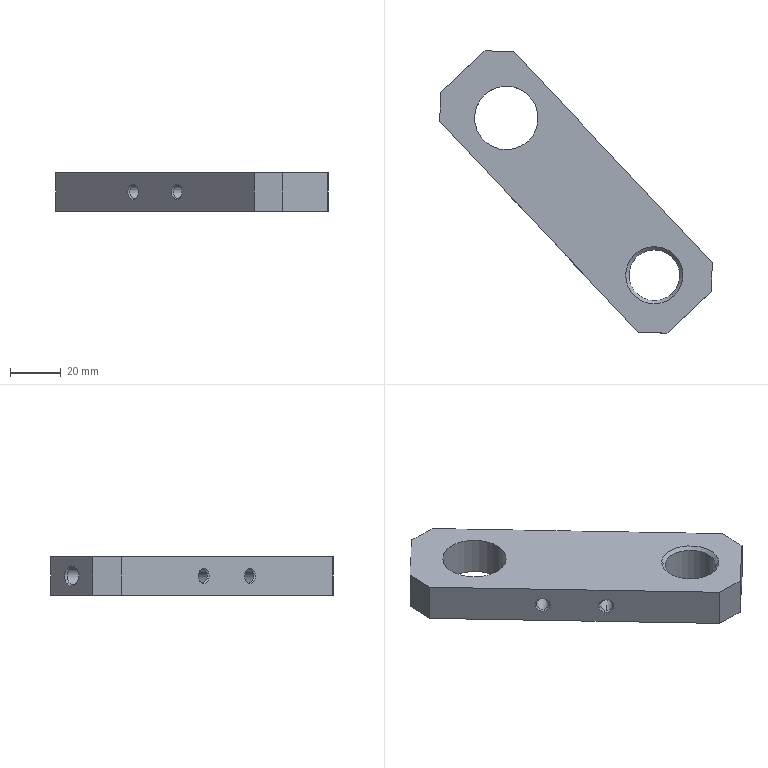Component | SolidWorks | LeftSupportBlock-1 | 1 solid | 32 faces | box 107.26 x 111.11 x 15 mm | volume 62679 mm3 | cone 12 | cylinder 10 | plane 10 | commonest cylinder face diameters 5 x4 6.8 x2 25 x2 20 x2
STEP:
#1=COLOUR_RGB('',0.7922,0.8196,0.9333);
#2=FILL_AREA_STYLE_COLOUR('',#1);
#3=FILL_AREA_STYLE('',(#2));
#4=SURFACE_STYLE_FILL_AREA(#3);
#5=SURFACE_SIDE_STYLE('',(#4));
#6=SURFACE_STYLE_USAGE(.BOTH.,#5);
#7=PRESENTATION_STYLE_ASSIGNMENT((#6));
#8=CARTESIAN_POINT('',(12.703,20.379,9.657));
#9=VERTEX_POINT('',#8);
#10=CARTESIAN_POINT('',(12.703,20.379,9.461));
#11=VERTEX_POINT('',#10);
#12=CARTESIAN_POINT('',(12.703,20.379,9.559));
#13=DIRECTION('',(-0.7282,-0.6854,-0.));
#14=DIRECTION('',(0.,0.,-1.));
#15=AXIS2_PLACEMENT_3D('',#12,#13,#14);
#16=CIRCLE('',#15,0.09843);
#17=EDGE_CURVE('',#9,#11,#16,.T.);
#18=ORIENTED_EDGE('',*,*,#17,.F.);
#19=CARTESIAN_POINT('',(12.688,20.365,9.678));
#20=VERTEX_POINT('',#19);
#21=CARTESIAN_POINT('',(12.688,20.365,9.678));
#22=DIRECTION('',(-0.5149,-0.4846,0.7071));
#23=VECTOR('',#22,39.37);
#24=LINE('',#21,#23);
#25=EDGE_CURVE('',#9,#20,#24,.T.);
#26=ORIENTED_EDGE('',*,*,#25,.T.);
#27=CARTESIAN_POINT('',(12.688,20.365,9.44));
#28=VERTEX_POINT('',#27);
#29=CARTESIAN_POINT('',(12.688,20.365,9.559));
#30=DIRECTION('',(-0.7282,-0.6854,-0.));
#31=DIRECTION('',(0.,0.,-1.));
#32=AXIS2_PLACEMENT_3D('',#29,#30,#31);
#33=CIRCLE('',#32,0.1191);
#34=EDGE_CURVE('',#20,#28,#33,.T.);
#35=ORIENTED_EDGE('',*,*,#34,.T.);
#36=CARTESIAN_POINT('',(12.688,20.365,9.44));
#37=DIRECTION('',(-0.5149,-0.4846,-0.7071));
#38=VECTOR('',#37,39.37);
#39=LINE('',#36,#38);
#40=EDGE_CURVE('',#11,#28,#39,.T.);
#41=ORIENTED_EDGE('',*,*,#40,.F.);
#42=EDGE_LOOP('',(#18,#26,#35,#41));
#43=FACE_OUTER_BOUND('',#42,.T.);
#44=CARTESIAN_POINT('',(12.688,20.365,9.559));
#45=DIRECTION('',(-0.7282,-0.6854,-0.));
#46=DIRECTION('',(0.,0.,-1.));
#47=AXIS2_PLACEMENT_3D('',#44,#45,#46);
#48=CONICAL_SURFACE('',#47,0.1191,0.7854);
#49=ADVANCED_FACE('',(#43),#48,.F.);
#50=CARTESIAN_POINT('',(13.262,20.905,9.657));
#51=VERTEX_POINT('',#50);
#52=CARTESIAN_POINT('',(13.262,20.905,9.461));
#53=VERTEX_POINT('',#52);
#54=CARTESIAN_POINT('',(13.262,20.905,9.559));
#55=DIRECTION('',(-0.7282,-0.6854,-0.));
#56=DIRECTION('',(0.,0.,-1.));
#57=AXIS2_PLACEMENT_3D('',#54,#55,#56);
#58=CIRCLE('',#57,0.09843);
#59=EDGE_CURVE('',#51,#53,#58,.T.);
#60=ORIENTED_EDGE('',*,*,#59,.F.);
#61=CARTESIAN_POINT('',(12.688,20.365,9.657));
#62=DIRECTION('',(-0.7282,-0.6854,-0.));
#63=VECTOR('',#62,39.37);
#64=LINE('',#61,#63);
#65=EDGE_CURVE('',#51,#9,#64,.T.);
#66=ORIENTED_EDGE('',*,*,#65,.T.);
#67=ORIENTED_EDGE('',*,*,#17,.T.);
#68=CARTESIAN_POINT('',(12.688,20.365,9.461));
#69=DIRECTION('',(-0.7282,-0.6854,-0.));
#70=VECTOR('',#69,39.37);
#71=LINE('',#68,#70);
#72=EDGE_CURVE('',#53,#11,#71,.T.);
#73=ORIENTED_EDGE('',*,*,#72,.F.);
#74=EDGE_LOOP('',(#60,#66,#67,#73));
#75=FACE_OUTER_BOUND('',#74,.T.);
#76=CARTESIAN_POINT('',(12.688,20.365,9.559));
#77=DIRECTION('',(-0.7282,-0.6854,-0.));
#78=DIRECTION('',(0.,0.,-1.));
#79=AXIS2_PLACEMENT_3D('',#76,#77,#78);
#80=CYLINDRICAL_SURFACE('',#79,0.09843);
#81=ADVANCED_FACE('',(#75),#80,.F.);
#82=CARTESIAN_POINT('',(13.305,20.945,9.559));
#83=VERTEX_POINT('',#82);
#84=CARTESIAN_POINT('',(13.262,20.905,9.461));
#85=DIRECTION('',(-0.375,-0.353,-0.8572));
#86=VECTOR('',#85,39.37);
#87=LINE('',#84,#86);
#88=EDGE_CURVE('',#83,#53,#87,.T.);
#89=ORIENTED_EDGE('',*,*,#88,.F.);
#90=CARTESIAN_POINT('',(13.262,20.905,9.657));
#91=DIRECTION('',(-0.375,-0.353,0.8572));
#92=VECTOR('',#91,39.37);
#93=LINE('',#90,#92);
#94=EDGE_CURVE('',#83,#51,#93,.T.);
#95=ORIENTED_EDGE('',*,*,#94,.T.);
#96=ORIENTED_EDGE('',*,*,#59,.T.);
#97=EDGE_LOOP('',(#89,#95,#96));
#98=FACE_OUTER_BOUND('',#97,.T.);
#99=CARTESIAN_POINT('',(13.262,20.905,9.559));
#100=DIRECTION('',(-0.7282,-0.6854,-0.));
#101=DIRECTION('',(0.,0.,-1.));
#102=AXIS2_PLACEMENT_3D('',#99,#100,#101);
#103=CONICAL_SURFACE('',#102,0.09843,1.03);
#104=ADVANCED_FACE('',(#98),#103,.F.);
#105=CARTESIAN_POINT('',(13.378,19.662,9.657));
#106=VERTEX_POINT('',#105);
#107=CARTESIAN_POINT('',(13.378,19.662,9.461));
#108=VERTEX_POINT('',#107);
#109=CARTESIAN_POINT('',(13.378,19.662,9.559));
#110=DIRECTION('',(-0.7282,-0.6854,-0.));
#111=DIRECTION('',(0.,0.,-1.));
#112=AXIS2_PLACEMENT_3D('',#109,#110,#111);
#113=CIRCLE('',#112,0.09843);
#114=EDGE_CURVE('',#106,#108,#113,.T.);
#115=ORIENTED_EDGE('',*,*,#114,.F.);
#116=CARTESIAN_POINT('',(13.363,19.648,9.678));
#117=VERTEX_POINT('',#116);
#118=CARTESIAN_POINT('',(13.363,19.648,9.678));
#119=DIRECTION('',(-0.5149,-0.4846,0.7071));
#120=VECTOR('',#119,39.37);
#121=LINE('',#118,#120);
#122=EDGE_CURVE('',#106,#117,#121,.T.);
#123=ORIENTED_EDGE('',*,*,#122,.T.);
#124=CARTESIAN_POINT('',(13.363,19.648,9.44));
#125=VERTEX_POINT('',#124);
#126=CARTESIAN_POINT('',(13.363,19.648,9.559));
#127=DIRECTION('',(-0.7282,-0.6854,-0.));
#128=DIRECTION('',(0.,0.,-1.));
#129=AXIS2_PLACEMENT_3D('',#126,#127,#128);
#130=CIRCLE('',#129,0.1191);
#131=EDGE_CURVE('',#117,#125,#130,.T.);
#132=ORIENTED_EDGE('',*,*,#131,.T.);
#133=CARTESIAN_POINT('',(13.363,19.648,9.44));
#134=DIRECTION('',(-0.5149,-0.4846,-0.7071));
#135=VECTOR('',#134,39.37);
#136=LINE('',#133,#135);
#137=EDGE_CURVE('',#108,#125,#136,.T.);
#138=ORIENTED_EDGE('',*,*,#137,.F.);
#139=EDGE_LOOP('',(#115,#123,#132,#138));
#140=FACE_OUTER_BOUND('',#139,.T.);
#141=CARTESIAN_POINT('',(13.363,19.648,9.559));
#142=DIRECTION('',(-0.7282,-0.6854,-0.));
#143=DIRECTION('',(0.,0.,-1.));
#144=AXIS2_PLACEMENT_3D('',#141,#142,#143);
#145=CONICAL_SURFACE('',#144,0.1191,0.7854);
#146=ADVANCED_FACE('',(#140),#145,.F.);
#147=CARTESIAN_POINT('',(13.936,20.188,9.657));
#148=VERTEX_POINT('',#147);
#149=CARTESIAN_POINT('',(13.936,20.188,9.461));
#150=VERTEX_POINT('',#149);
#151=CARTESIAN_POINT('',(13.936,20.188,9.559));
#152=DIRECTION('',(-0.7282,-0.6854,-0.));
#153=DIRECTION('',(0.,0.,-1.));
#154=AXIS2_PLACEMENT_3D('',#151,#152,#153);
#155=CIRCLE('',#154,0.09843);
#156=EDGE_CURVE('',#148,#150,#155,.T.);
#157=ORIENTED_EDGE('',*,*,#156,.F.);
#158=CARTESIAN_POINT('',(13.363,19.648,9.657));
#159=DIRECTION('',(-0.7282,-0.6854,-0.));
#160=VECTOR('',#159,39.37);
#161=LINE('',#158,#160);
#162=EDGE_CURVE('',#148,#106,#161,.T.);
#163=ORIENTED_EDGE('',*,*,#162,.T.);
#164=ORIENTED_EDGE('',*,*,#114,.T.);
#165=CARTESIAN_POINT('',(13.363,19.648,9.461));
#166=DIRECTION('',(-0.7282,-0.6854,-0.));
#167=VECTOR('',#166,39.37);
#168=LINE('',#165,#167);
#169=EDGE_CURVE('',#150,#108,#168,.T.);
#170=ORIENTED_EDGE('',*,*,#169,.F.);
#171=EDGE_LOOP('',(#157,#163,#164,#170));
#172=FACE_OUTER_BOUND('',#171,.T.);
#173=CARTESIAN_POINT('',(13.363,19.648,9.559));
#174=DIRECTION('',(-0.7282,-0.6854,-0.));
#175=DIRECTION('',(0.,0.,-1.));
#176=AXIS2_PLACEMENT_3D('',#173,#174,#175);
#177=CYLINDRICAL_SURFACE('',#176,0.09843);
#178=ADVANCED_FACE('',(#172),#177,.F.);
#179=CARTESIAN_POINT('',(13.979,20.228,9.559));
#180=VERTEX_POINT('',#179);
#181=CARTESIAN_POINT('',(13.936,20.188,9.461));
#182=DIRECTION('',(-0.375,-0.353,-0.8572));
#183=VECTOR('',#182,39.37);
#184=LINE('',#181,#183);
#185=EDGE_CURVE('',#180,#150,#184,.T.);
#186=ORIENTED_EDGE('',*,*,#185,.F.);
#187=CARTESIAN_POINT('',(13.936,20.188,9.657));
#188=DIRECTION('',(-0.375,-0.353,0.8572));
#189=VECTOR('',#188,39.37);
#190=LINE('',#187,#189);
#191=EDGE_CURVE('',#180,#148,#190,.T.);
#192=ORIENTED_EDGE('',*,*,#191,.T.);
#193=ORIENTED_EDGE('',*,*,#156,.T.);
#194=EDGE_LOOP('',(#186,#192,#193));
#195=FACE_OUTER_BOUND('',#194,.T.);
#196=CARTESIAN_POINT('',(13.936,20.188,9.559));
#197=DIRECTION('',(-0.7282,-0.6854,-0.));
#198=DIRECTION('',(0.,0.,-1.));
#199=AXIS2_PLACEMENT_3D('',#196,#197,#198);
#200=CONICAL_SURFACE('',#199,0.09843,1.03);
#201=ADVANCED_FACE('',(#195),#200,.F.);
#202=CARTESIAN_POINT('',(11.862,22.392,9.425));
#203=VERTEX_POINT('',#202);
#204=CARTESIAN_POINT('',(11.862,22.392,9.693));
#205=VERTEX_POINT('',#204);
#206=CARTESIAN_POINT('',(11.862,22.392,9.559));
#207=DIRECTION('',(-0.6854,0.7282,-0.));
#208=DIRECTION('',(0.,0.,1.));
#209=AXIS2_PLACEMENT_3D('',#206,#207,#208);
#210=CIRCLE('',#209,0.1339);
#211=EDGE_CURVE('',#203,#205,#210,.T.);
#212=ORIENTED_EDGE('',*,*,#211,.F.);
#213=CARTESIAN_POINT('',(11.845,22.41,9.401));
#214=VERTEX_POINT('',#213);
#215=CARTESIAN_POINT('',(11.845,22.41,9.401));
#216=DIRECTION('',(-0.4846,0.5149,-0.7071));
#217=VECTOR('',#216,39.37);
#218=LINE('',#215,#217);
#219=EDGE_CURVE('',#203,#214,#218,.T.);
#220=ORIENTED_EDGE('',*,*,#219,.T.);
#221=CARTESIAN_POINT('',(11.845,22.41,9.718));
#222=VERTEX_POINT('',#221);
#223=CARTESIAN_POINT('',(11.845,22.41,9.559));
#224=DIRECTION('',(-0.6854,0.7282,-0.));
#225=DIRECTION('',(0.,0.,1.));
#226=AXIS2_PLACEMENT_3D('',#223,#224,#225);
#227=CIRCLE('',#226,0.1585);
#228=EDGE_CURVE('',#214,#222,#227,.T.);
#229=ORIENTED_EDGE('',*,*,#228,.T.);
#230=CARTESIAN_POINT('',(11.845,22.41,9.718));
#231=DIRECTION('',(-0.4846,0.5149,0.7071));
#232=VECTOR('',#231,39.37);
#233=LINE('',#230,#232);
#234=EDGE_CURVE('',#205,#222,#233,.T.);
#235=ORIENTED_EDGE('',*,*,#234,.F.);
#236=EDGE_LOOP('',(#212,#220,#229,#235));
#237=FACE_OUTER_BOUND('',#236,.T.);
#238=CARTESIAN_POINT('',(11.845,22.41,9.559));
#239=DIRECTION('',(-0.6854,0.7282,-0.));
#240=DIRECTION('',(0.,0.,1.));
#241=AXIS2_PLACEMENT_3D('',#238,#239,#240);
#242=CONICAL_SURFACE('',#241,0.1585,0.7854);
#243=ADVANCED_FACE('',(#237),#242,.F.);
#244=CARTESIAN_POINT('',(12.182,22.051,9.425));
#245=VERTEX_POINT('',#244);
#246=CARTESIAN_POINT('',(12.182,22.051,9.693));
#247=VERTEX_POINT('',#246);
#248=CARTESIAN_POINT('',(12.182,22.051,9.425));
#249=CARTESIAN_POINT('',(12.176,22.045,9.425));
#250=CARTESIAN_POINT('',(12.17,22.039,9.426));
#251=CARTESIAN_POINT('',(12.158,22.027,9.43));
#252=CARTESIAN_POINT('',(12.152,22.02,9.432));
#253=CARTESIAN_POINT('',(12.142,22.008,9.439));
#254=CARTESIAN_POINT('',(12.137,22.002,9.443));
#255=CARTESIAN_POINT('',(12.128,21.99,9.453));
#256=CARTESIAN_POINT('',(12.123,21.985,9.458));
#257=CARTESIAN_POINT('',(12.116,21.975,9.471));
#258=CARTESIAN_POINT('',(12.113,21.97,9.477));
#259=CARTESIAN_POINT('',(12.107,21.962,9.492));
#260=CARTESIAN_POINT('',(12.105,21.958,9.499));
#261=CARTESIAN_POINT('',(12.101,21.952,9.516));
#262=CARTESIAN_POINT('',(12.1,21.95,9.524));
#263=CARTESIAN_POINT('',(12.098,21.947,9.541));
#264=CARTESIAN_POINT('',(12.098,21.946,9.55));
#265=CARTESIAN_POINT('',(12.098,21.946,9.568));
#266=CARTESIAN_POINT('',(12.098,21.947,9.577));
#267=CARTESIAN_POINT('',(12.1,21.95,9.594));
#268=CARTESIAN_POINT('',(12.101,21.952,9.602));
#269=CARTESIAN_POINT('',(12.105,21.958,9.618));
#270=CARTESIAN_POINT('',(12.107,21.962,9.626));
#271=CARTESIAN_POINT('',(12.113,21.97,9.641));
#272=CARTESIAN_POINT('',(12.116,21.975,9.648));
#273=CARTESIAN_POINT('',(12.123,21.985,9.66));
#274=CARTESIAN_POINT('',(12.128,21.99,9.665));
#275=CARTESIAN_POINT('',(12.137,22.002,9.675));
#276=CARTESIAN_POINT('',(12.141,22.008,9.679));
#277=CARTESIAN_POINT('',(12.152,22.02,9.686));
#278=CARTESIAN_POINT('',(12.158,22.027,9.689));
#279=CARTESIAN_POINT('',(12.17,22.039,9.692));
#280=CARTESIAN_POINT('',(12.176,22.045,9.693));
#281=CARTESIAN_POINT('',(12.182,22.051,9.693));
#282=B_SPLINE_CURVE_WITH_KNOTS('',3,(#248,#249,#250,#251,#252,#253,#254,#255,#256,#257,#258,#259,#260,#261,#262,#263,#264,#265,#266,#267,#268,#269,#270,#271,#272,#273,#274,#275,#276,#277,#278,#279,#280,#281),.UNSPECIFIED.,.F.,.F.,(4,2,2,2,2,2,2,2,2,2,2,2,2,2,2,2,4),(0.01068,0.01135,0.01202,0.01268,0.01335,0.01402,0.01468,0.01535,0.01602,0.01669,0.01735,0.01802,0.01869,0.01936,0.02002,0.02069,0.02136),.UNSPECIFIED.);
#283=EDGE_CURVE('',#245,#247,#282,.T.);
#284=ORIENTED_EDGE('',*,*,#283,.F.);
#285=CARTESIAN_POINT('',(11.845,22.41,9.425));
#286=DIRECTION('',(-0.6854,0.7282,-0.));
#287=VECTOR('',#286,39.37);
#288=LINE('',#285,#287);
#289=EDGE_CURVE('',#245,#203,#288,.T.);
#290=ORIENTED_EDGE('',*,*,#289,.T.);
#291=ORIENTED_EDGE('',*,*,#211,.T.);
#292=CARTESIAN_POINT('',(11.845,22.41,9.693));
#293=DIRECTION('',(-0.6854,0.7282,-0.));
#294=VECTOR('',#293,39.37);
#295=LINE('',#292,#294);
#296=EDGE_CURVE('',#247,#205,#295,.T.);
#297=ORIENTED_EDGE('',*,*,#296,.F.);
#298=EDGE_LOOP('',(#284,#290,#291,#297));
#299=FACE_OUTER_BOUND('',#298,.T.);
#300=CARTESIAN_POINT('',(11.845,22.41,9.559));
#301=DIRECTION('',(-0.6854,0.7282,-0.));
#302=DIRECTION('',(0.,0.,1.));
#303=AXIS2_PLACEMENT_3D('',#300,#301,#302);
#304=CYLINDRICAL_SURFACE('',#303,0.1339);
#305=ADVANCED_FACE('',(#299),#304,.F.);
#306=CARTESIAN_POINT('',(12.857,21.335,9.854));
#307=VERTEX_POINT('',#306);
#308=CARTESIAN_POINT('',(12.182,22.051,9.854));
#309=VERTEX_POINT('',#308);
#310=CARTESIAN_POINT('',(12.52,21.693,9.854));
#311=DIRECTION('',(0.,-0.,-1.));
#312=DIRECTION('',(-0.6854,0.7282,0.));
#313=AXIS2_PLACEMENT_3D('',#310,#311,#312);
#314=CIRCLE('',#313,0.4921);
#315=EDGE_CURVE('',#307,#309,#314,.T.);
#316=ORIENTED_EDGE('',*,*,#315,.F.);
#317=CARTESIAN_POINT('',(12.857,21.335,9.264));
#318=VERTEX_POINT('',#317);
#319=CARTESIAN_POINT('',(12.857,21.335,9.264));
#320=DIRECTION('',(0.,-0.,-1.));
#321=VECTOR('',#320,39.37);
#322=LINE('',#319,#321);
#323=EDGE_CURVE('',#307,#318,#322,.T.);
#324=ORIENTED_EDGE('',*,*,#323,.T.);
#325=CARTESIAN_POINT('',(12.182,22.051,9.264));
#326=VERTEX_POINT('',#325);
#327=CARTESIAN_POINT('',(12.52,21.693,9.264));
#328=DIRECTION('',(0.,-0.,-1.));
#329=DIRECTION('',(-0.6854,0.7282,0.));
#330=AXIS2_PLACEMENT_3D('',#327,#328,#329);
#331=CIRCLE('',#330,0.4921);
#332=EDGE_CURVE('',#318,#326,#331,.T.);
#333=ORIENTED_EDGE('',*,*,#332,.T.);
#334=CARTESIAN_POINT('',(12.182,22.051,9.264));
#335=DIRECTION('',(0.,-0.,-1.));
#336=VECTOR('',#335,39.37);
#337=LINE('',#334,#336);
#338=EDGE_CURVE('',#245,#326,#337,.T.);
#339=ORIENTED_EDGE('',*,*,#338,.F.);
#340=ORIENTED_EDGE('',*,*,#283,.T.);
#341=CARTESIAN_POINT('',(12.182,22.051,9.264));
#342=DIRECTION('',(0.,-0.,-1.));
#343=VECTOR('',#342,39.37);
#344=LINE('',#341,#343);
#345=EDGE_CURVE('',#309,#247,#344,.T.);
#346=ORIENTED_EDGE('',*,*,#345,.F.);
#347=EDGE_LOOP('',(#316,#324,#333,#339,#340,#346));
#348=FACE_OUTER_BOUND('',#347,.T.);
#349=CARTESIAN_POINT('',(12.52,21.693,9.264));
#350=DIRECTION('',(0.,-0.,-1.));
#351=DIRECTION('',(-0.6854,0.7282,0.));
#352=AXIS2_PLACEMENT_3D('',#349,#350,#351);
#353=CYLINDRICAL_SURFACE('',#352,0.4921);
#354=ADVANCED_FACE('',(#348),#353,.F.);
#355=CARTESIAN_POINT('',(14.543,19.543,9.804));
#356=VERTEX_POINT('',#355);
#357=CARTESIAN_POINT('',(15.083,18.969,9.804));
#358=VERTEX_POINT('',#357);
#359=CARTESIAN_POINT('',(14.813,19.256,9.804));
#360=DIRECTION('',(-0.,0.,1.));
#361=DIRECTION('',(0.6854,-0.7282,0.));
#362=AXIS2_PLACEMENT_3D('',#359,#360,#361);
#363=CIRCLE('',#362,0.3937);
#364=EDGE_CURVE('',#356,#358,#363,.T.);
#365=ORIENTED_EDGE('',*,*,#364,.F.);
#366=CARTESIAN_POINT('',(14.509,19.579,9.854));
#367=VERTEX_POINT('',#366);
#368=CARTESIAN_POINT('',(14.509,19.579,9.854));
#369=DIRECTION('',(-0.4846,0.5149,0.7071));
#370=VECTOR('',#369,39.37);
#371=LINE('',#368,#370);
#372=EDGE_CURVE('',#356,#367,#371,.T.);
#373=ORIENTED_EDGE('',*,*,#372,.T.);
#374=CARTESIAN_POINT('',(15.118,18.933,9.854));
#375=VERTEX_POINT('',#374);
#376=CARTESIAN_POINT('',(14.813,19.256,9.854));
#377=DIRECTION('',(-0.,0.,1.));
#378=DIRECTION('',(0.6854,-0.7282,0.));
#379=AXIS2_PLACEMENT_3D('',#376,#377,#378);
#380=CIRCLE('',#379,0.4439);
#381=EDGE_CURVE('',#367,#375,#380,.T.);
#382=ORIENTED_EDGE('',*,*,#381,.T.);
#383=CARTESIAN_POINT('',(15.118,18.933,9.854));
#384=DIRECTION('',(0.4846,-0.5149,0.7071));
#385=VECTOR('',#384,39.37);
#386=LINE('',#383,#385);
#387=EDGE_CURVE('',#358,#375,#386,.T.);
#388=ORIENTED_EDGE('',*,*,#387,.F.);
#389=EDGE_LOOP('',(#365,#373,#382,#388));
#390=FACE_OUTER_BOUND('',#389,.T.);
#391=CARTESIAN_POINT('',(14.813,19.256,9.854));
#392=DIRECTION('',(-0.,0.,1.));
#393=DIRECTION('',(0.6854,-0.7282,0.));
#394=AXIS2_PLACEMENT_3D('',#391,#392,#393);
#395=CONICAL_SURFACE('',#394,0.4439,0.7854);
#396=ADVANCED_FACE('',(#390),#395,.F.);
#397=CARTESIAN_POINT('',(14.543,19.543,9.264));
#398=VERTEX_POINT('',#397);
#399=CARTESIAN_POINT('',(15.083,18.969,9.264));
#400=VERTEX_POINT('',#399);
#401=CARTESIAN_POINT('',(14.813,19.256,9.264));
#402=DIRECTION('',(-0.,0.,1.));
#403=DIRECTION('',(0.6854,-0.7282,0.));
#404=AXIS2_PLACEMENT_3D('',#401,#402,#403);
#405=CIRCLE('',#404,0.3937);
#406=EDGE_CURVE('',#398,#400,#405,.T.);
#407=ORIENTED_EDGE('',*,*,#406,.F.);
#408=CARTESIAN_POINT('',(14.543,19.543,9.854));
#409=DIRECTION('',(-0.,0.,1.));
#410=VECTOR('',#409,39.37);
#411=LINE('',#408,#410);
#412=EDGE_CURVE('',#398,#356,#411,.T.);
#413=ORIENTED_EDGE('',*,*,#412,.T.);
#414=ORIENTED_EDGE('',*,*,#364,.T.);
#415=CARTESIAN_POINT('',(15.083,18.969,9.854));
#416=DIRECTION('',(-0.,0.,1.));
#417=VECTOR('',#416,39.37);
#418=LINE('',#415,#417);
#419=EDGE_CURVE('',#400,#358,#418,.T.);
#420=ORIENTED_EDGE('',*,*,#419,.F.);
#421=EDGE_LOOP('',(#407,#413,#414,#420));
#422=FACE_OUTER_BOUND('',#421,.T.);
#423=CARTESIAN_POINT('',(14.813,19.256,9.854));
#424=DIRECTION('',(-0.,0.,1.));
#425=DIRECTION('',(0.6854,-0.7282,0.));
#426=AXIS2_PLACEMENT_3D('',#423,#424,#425);
#427=CYLINDRICAL_SURFACE('',#426,0.3937);
#428=ADVANCED_FACE('',(#422),#427,.F.);
#429=CARTESIAN_POINT('',(12.634,22.72,9.854));
#430=VERTEX_POINT('',#429);
#431=CARTESIAN_POINT('',(12.189,22.733,9.854));
#432=VERTEX_POINT('',#431);
#433=CARTESIAN_POINT('',(12.634,22.72,9.854));
#434=DIRECTION('',(-0.9995,0.03026,-0.));
#435=VECTOR('',#434,39.37);
#436=LINE('',#433,#435);
#437=EDGE_CURVE('',#430,#432,#436,.T.);
#438=ORIENTED_EDGE('',*,*,#437,.F.);
#439=CARTESIAN_POINT('',(12.634,22.72,9.264));
#440=VERTEX_POINT('',#439);
#441=CARTESIAN_POINT('',(12.634,22.72,9.264));
#442=DIRECTION('',(-0.,0.,1.));
#443=VECTOR('',#442,39.37);
#444=LINE('',#441,#443);
#445=EDGE_CURVE('',#440,#430,#444,.T.);
#446=ORIENTED_EDGE('',*,*,#445,.F.);
#447=CARTESIAN_POINT('',(12.189,22.733,9.264));
#448=VERTEX_POINT('',#447);
#449=CARTESIAN_POINT('',(12.634,22.72,9.264));
#450=DIRECTION('',(-0.9995,0.03026,-0.));
#451=VECTOR('',#450,39.37);
#452=LINE('',#449,#451);
#453=EDGE_CURVE('',#440,#448,#452,.T.);
#454=ORIENTED_EDGE('',*,*,#453,.T.);
#455=CARTESIAN_POINT('',(12.189,22.733,9.264));
#456=DIRECTION('',(-0.,0.,1.));
#457=VECTOR('',#456,39.37);
#458=LINE('',#455,#457);
#459=EDGE_CURVE('',#448,#432,#458,.T.);
#460=ORIENTED_EDGE('',*,*,#459,.T.);
#461=EDGE_LOOP('',(#438,#446,#454,#460));
#462=FACE_OUTER_BOUND('',#461,.T.);
#463=CARTESIAN_POINT('',(12.634,22.72,9.264));
#464=DIRECTION('',(0.03026,0.9995,-0.));
#465=DIRECTION('',(-0.9995,0.03026,-0.));
#466=AXIS2_PLACEMENT_3D('',#463,#464,#465);
#467=PLANE('',#466);
#468=ADVANCED_FACE('',(#462),#467,.T.);
#469=CARTESIAN_POINT('',(15.71,19.452,9.854));
#470=VERTEX_POINT('',#469);
#471=CARTESIAN_POINT('',(15.71,19.452,9.854));
#472=DIRECTION('',(-0.6854,0.7282,-0.));
#473=VECTOR('',#472,39.37);
#474=LINE('',#471,#473);
#475=EDGE_CURVE('',#470,#430,#474,.T.);
#476=ORIENTED_EDGE('',*,*,#475,.F.);
#477=CARTESIAN_POINT('',(15.71,19.452,9.264));
#478=VERTEX_POINT('',#477);
#479=CARTESIAN_POINT('',(15.71,19.452,9.264));
#480=DIRECTION('',(-0.,0.,1.));
#481=VECTOR('',#480,39.37);
#482=LINE('',#479,#481);
#483=EDGE_CURVE('',#478,#470,#482,.T.);
#484=ORIENTED_EDGE('',*,*,#483,.F.);
#485=CARTESIAN_POINT('',(15.71,19.452,9.264));
#486=DIRECTION('',(-0.6854,0.7282,-0.));
#487=VECTOR('',#486,39.37);
#488=LINE('',#485,#487);
#489=EDGE_CURVE('',#478,#440,#488,.T.);
#490=ORIENTED_EDGE('',*,*,#489,.T.);
#491=ORIENTED_EDGE('',*,*,#445,.T.);
#492=EDGE_LOOP('',(#476,#484,#490,#491));
#493=FACE_OUTER_BOUND('',#492,.T.);
#494=CARTESIAN_POINT('',(15.71,19.452,9.264));
#495=DIRECTION('',(0.7282,0.6854,0.));
#496=DIRECTION('',(-0.,0.,1.));
#497=AXIS2_PLACEMENT_3D('',#494,#495,#496);
#498=PLANE('',#497);
#499=ADVANCED_FACE('',(#493),#498,.T.);
#500=CARTESIAN_POINT('',(15.697,19.007,9.854));
#501=VERTEX_POINT('',#500);
#502=CARTESIAN_POINT('',(15.697,19.007,9.854));
#503=DIRECTION('',(0.03026,0.9995,-0.));
#504=VECTOR('',#503,39.37);
#505=LINE('',#502,#504);
#506=EDGE_CURVE('',#501,#470,#505,.T.);
#507=ORIENTED_EDGE('',*,*,#506,.F.);
#508=CARTESIAN_POINT('',(15.697,19.007,9.264));
#509=VERTEX_POINT('',#508);
#510=CARTESIAN_POINT('',(15.697,19.007,9.264));
#511=DIRECTION('',(-0.,0.,1.));
#512=VECTOR('',#511,39.37);
#513=LINE('',#510,#512);
#514=EDGE_CURVE('',#509,#501,#513,.T.);
#515=ORIENTED_EDGE('',*,*,#514,.F.);
#516=CARTESIAN_POINT('',(15.697,19.007,9.264));
#517=DIRECTION('',(0.03026,0.9995,-0.));
#518=VECTOR('',#517,39.37);
#519=LINE('',#516,#518);
#520=EDGE_CURVE('',#509,#478,#519,.T.);
#521=ORIENTED_EDGE('',*,*,#520,.T.);
#522=ORIENTED_EDGE('',*,*,#483,.T.);
#523=EDGE_LOOP('',(#507,#515,#521,#522));
#524=FACE_OUTER_BOUND('',#523,.T.);
#525=CARTESIAN_POINT('',(15.697,19.007,9.264));
#526=DIRECTION('',(0.9995,-0.03026,0.));
#527=DIRECTION('',(0.03026,0.9995,-0.));
#528=AXIS2_PLACEMENT_3D('',#525,#526,#527);
#529=PLANE('',#528);
#530=ADVANCED_FACE('',(#524),#529,.T.);
#531=CARTESIAN_POINT('',(15.009,18.359,9.854));
#532=VERTEX_POINT('',#531);
#533=CARTESIAN_POINT('',(15.009,18.359,9.854));
#534=DIRECTION('',(0.7282,0.6854,0.));
#535=VECTOR('',#534,39.37);
#536=LINE('',#533,#535);
#537=EDGE_CURVE('',#532,#501,#536,.T.);
#538=ORIENTED_EDGE('',*,*,#537,.F.);
#539=CARTESIAN_POINT('',(15.009,18.359,9.264));
#540=VERTEX_POINT('',#539);
#541=CARTESIAN_POINT('',(15.009,18.359,9.264));
#542=DIRECTION('',(-0.,0.,1.));
#543=VECTOR('',#542,39.37);
#544=LINE('',#541,#543);
#545=EDGE_CURVE('',#540,#532,#544,.T.);
#546=ORIENTED_EDGE('',*,*,#545,.F.);
#547=CARTESIAN_POINT('',(15.009,18.359,9.264));
#548=DIRECTION('',(0.7282,0.6854,0.));
#549=VECTOR('',#548,39.37);
#550=LINE('',#547,#549);
#551=EDGE_CURVE('',#540,#509,#550,.T.);
#552=ORIENTED_EDGE('',*,*,#551,.T.);
#553=ORIENTED_EDGE('',*,*,#514,.T.);
#554=EDGE_LOOP('',(#538,#546,#552,#553));
#555=FACE_OUTER_BOUND('',#554,.T.);
#556=CARTESIAN_POINT('',(15.009,18.359,9.264));
#557=DIRECTION('',(0.6854,-0.7282,0.));
#558=DIRECTION('',(0.,-0.,-1.));
#559=AXIS2_PLACEMENT_3D('',#556,#557,#558);
#560=PLANE('',#559);
#561=ADVANCED_FACE('',(#555),#560,.T.);
#562=CARTESIAN_POINT('',(14.564,18.372,9.854));
#563=VERTEX_POINT('',#562);
#564=CARTESIAN_POINT('',(14.564,18.372,9.854));
#565=DIRECTION('',(0.9995,-0.03026,0.));
#566=VECTOR('',#565,39.37);
#567=LINE('',#564,#566);
#568=EDGE_CURVE('',#563,#532,#567,.T.);
#569=ORIENTED_EDGE('',*,*,#568,.F.);
#570=CARTESIAN_POINT('',(14.564,18.372,9.264));
#571=VERTEX_POINT('',#570);
#572=CARTESIAN_POINT('',(14.564,18.372,9.264));
#573=DIRECTION('',(-0.,0.,1.));
#574=VECTOR('',#573,39.37);
#575=LINE('',#572,#574);
#576=EDGE_CURVE('',#571,#563,#575,.T.);
#577=ORIENTED_EDGE('',*,*,#576,.F.);
#578=CARTESIAN_POINT('',(14.564,18.372,9.264));
#579=DIRECTION('',(0.9995,-0.03026,0.));
#580=VECTOR('',#579,39.37);
#581=LINE('',#578,#580);
#582=EDGE_CURVE('',#571,#540,#581,.T.);
#583=ORIENTED_EDGE('',*,*,#582,.T.);
#584=ORIENTED_EDGE('',*,*,#545,.T.);
#585=EDGE_LOOP('',(#569,#577,#583,#584));
#586=FACE_OUTER_BOUND('',#585,.T.);
#587=CARTESIAN_POINT('',(14.564,18.372,9.264));
#588=DIRECTION('',(-0.03026,-0.9995,0.));
#589=DIRECTION('',(0.9995,-0.03026,0.));
#590=AXIS2_PLACEMENT_3D('',#587,#588,#589);
#591=PLANE('',#590);
#592=ADVANCED_FACE('',(#586),#591,.T.);
#593=CARTESIAN_POINT('',(12.688,20.365,9.559));
#594=DIRECTION('',(-0.7282,-0.6854,-0.));
#595=DIRECTION('',(0.,0.,-1.));
#596=AXIS2_PLACEMENT_3D('',#593,#594,#595);
#597=CIRCLE('',#596,0.1191);
#598=EDGE_CURVE('',#28,#20,#597,.T.);
#599=ORIENTED_EDGE('',*,*,#598,.F.);
#600=ORIENTED_EDGE('',*,*,#34,.F.);
#601=EDGE_LOOP('',(#599,#600));
#602=FACE_BOUND('',#601,.T.);
#603=CARTESIAN_POINT('',(13.363,19.648,9.559));
#604=DIRECTION('',(-0.7282,-0.6854,-0.));
#605=DIRECTION('',(0.,0.,-1.));
#606=AXIS2_PLACEMENT_3D('',#603,#604,#605);
#607=CIRCLE('',#606,0.1191);
#608=EDGE_CURVE('',#125,#117,#607,.T.);
#609=ORIENTED_EDGE('',*,*,#608,.F.);
#610=ORIENTED_EDGE('',*,*,#131,.F.);
#611=EDGE_LOOP('',(#609,#610));
#612=FACE_BOUND('',#611,.T.);
#613=CARTESIAN_POINT('',(11.488,21.641,9.854));
#614=VERTEX_POINT('',#613);
#615=CARTESIAN_POINT('',(11.488,21.641,9.854));
#616=DIRECTION('',(0.6854,-0.7282,0.));
#617=VECTOR('',#616,39.37);
#618=LINE('',#615,#617);
#619=EDGE_CURVE('',#614,#563,#618,.T.);
#620=ORIENTED_EDGE('',*,*,#619,.F.);
#621=CARTESIAN_POINT('',(11.488,21.641,9.264));
#622=VERTEX_POINT('',#621);
#623=CARTESIAN_POINT('',(11.488,21.641,9.264));
#624=DIRECTION('',(-0.,0.,1.));
#625=VECTOR('',#624,39.37);
#626=LINE('',#623,#625);
#627=EDGE_CURVE('',#622,#614,#626,.T.);
#628=ORIENTED_EDGE('',*,*,#627,.F.);
#629=CARTESIAN_POINT('',(11.488,21.641,9.264));
#630=DIRECTION('',(0.6854,-0.7282,0.));
#631=VECTOR('',#630,39.37);
#632=LINE('',#629,#631);
#633=EDGE_CURVE('',#622,#571,#632,.T.);
#634=ORIENTED_EDGE('',*,*,#633,.T.);
#635=ORIENTED_EDGE('',*,*,#576,.T.);
#636=EDGE_LOOP('',(#620,#628,#634,#635));
#637=FACE_OUTER_BOUND('',#636,.T.);
#638=CARTESIAN_POINT('',(11.488,21.641,9.264));
#639=DIRECTION('',(-0.7282,-0.6854,-0.));
#640=DIRECTION('',(0.6854,-0.7282,0.));
#641=AXIS2_PLACEMENT_3D('',#638,#639,#640);
#642=PLANE('',#641);
#643=ADVANCED_FACE('',(#602,#612,#637),#642,.T.);
#644=CARTESIAN_POINT('',(11.501,22.086,9.854));
#645=VERTEX_POINT('',#644);
#646=CARTESIAN_POINT('',(11.501,22.086,9.854));
#647=DIRECTION('',(-0.03026,-0.9995,0.));
#648=VECTOR('',#647,39.37);
#649=LINE('',#646,#648);
#650=EDGE_CURVE('',#645,#614,#649,.T.);
#651=ORIENTED_EDGE('',*,*,#650,.F.);
#652=CARTESIAN_POINT('',(11.501,22.086,9.264));
#653=VERTEX_POINT('',#652);
#654=CARTESIAN_POINT('',(11.501,22.086,9.264));
#655=DIRECTION('',(-0.,0.,1.));
#656=VECTOR('',#655,39.37);
#657=LINE('',#654,#656);
#658=EDGE_CURVE('',#653,#645,#657,.T.);
#659=ORIENTED_EDGE('',*,*,#658,.F.);
#660=CARTESIAN_POINT('',(11.501,22.086,9.264));
#661=DIRECTION('',(-0.03026,-0.9995,0.));
#662=VECTOR('',#661,39.37);
#663=LINE('',#660,#662);
#664=EDGE_CURVE('',#653,#622,#663,.T.);
#665=ORIENTED_EDGE('',*,*,#664,.T.);
#666=ORIENTED_EDGE('',*,*,#627,.T.);
#667=EDGE_LOOP('',(#651,#659,#665,#666));
#668=FACE_OUTER_BOUND('',#667,.T.);
#669=CARTESIAN_POINT('',(11.501,22.086,9.264));
#670=DIRECTION('',(-0.9995,0.03026,-0.));
#671=DIRECTION('',(-0.03026,-0.9995,0.));
#672=AXIS2_PLACEMENT_3D('',#669,#670,#671);
#673=PLANE('',#672);
#674=ADVANCED_FACE('',(#668),#673,.T.);
#675=CARTESIAN_POINT('',(11.845,22.41,9.559));
#676=DIRECTION('',(-0.6854,0.7282,-0.));
#677=DIRECTION('',(0.,0.,1.));
#678=AXIS2_PLACEMENT_3D('',#675,#676,#677);
#679=CIRCLE('',#678,0.1585);
#680=EDGE_CURVE('',#222,#214,#679,.T.);
#681=ORIENTED_EDGE('',*,*,#680,.F.);
#682=ORIENTED_EDGE('',*,*,#228,.F.);
#683=EDGE_LOOP('',(#681,#682));
#684=FACE_BOUND('',#683,.T.);
#685=CARTESIAN_POINT('',(12.189,22.733,9.854));
#686=DIRECTION('',(-0.7282,-0.6854,-0.));
#687=VECTOR('',#686,39.37);
#688=LINE('',#685,#687);
#689=EDGE_CURVE('',#432,#645,#688,.T.);
#690=ORIENTED_EDGE('',*,*,#689,.F.);
#691=ORIENTED_EDGE('',*,*,#459,.F.);
#692=CARTESIAN_POINT('',(12.189,22.733,9.264));
#693=DIRECTION('',(-0.7282,-0.6854,-0.));
#694=VECTOR('',#693,39.37);
#695=LINE('',#692,#694);
#696=EDGE_CURVE('',#448,#653,#695,.T.);
#697=ORIENTED_EDGE('',*,*,#696,.T.);
#698=ORIENTED_EDGE('',*,*,#658,.T.);
#699=EDGE_LOOP('',(#690,#691,#697,#698));
#700=FACE_OUTER_BOUND('',#699,.T.);
#701=CARTESIAN_POINT('',(12.189,22.733,9.264));
#702=DIRECTION('',(-0.6854,0.7282,-0.));
#703=DIRECTION('',(-0.,0.,1.));
#704=AXIS2_PLACEMENT_3D('',#701,#702,#703);
#705=PLANE('',#704);
#706=ADVANCED_FACE('',(#684,#700),#705,.T.);
#707=CARTESIAN_POINT('',(12.52,21.693,9.264));
#708=DIRECTION('',(0.,-0.,-1.));
#709=DIRECTION('',(-0.6854,0.7282,0.));
#710=AXIS2_PLACEMENT_3D('',#707,#708,#709);
#711=CIRCLE('',#710,0.4921);
#712=EDGE_CURVE('',#326,#318,#711,.T.);
#713=ORIENTED_EDGE('',*,*,#712,.F.);
#714=ORIENTED_EDGE('',*,*,#332,.F.);
#715=EDGE_LOOP('',(#713,#714));
#716=FACE_BOUND('',#715,.T.);
#717=CARTESIAN_POINT('',(14.813,19.256,9.264));
#718=DIRECTION('',(-0.,0.,1.));
#719=DIRECTION('',(0.6854,-0.7282,0.));
#720=AXIS2_PLACEMENT_3D('',#717,#718,#719);
#721=CIRCLE('',#720,0.3937);
#722=EDGE_CURVE('',#400,#398,#721,.T.);
#723=ORIENTED_EDGE('',*,*,#722,.T.);
#724=ORIENTED_EDGE('',*,*,#406,.T.);
#725=EDGE_LOOP('',(#723,#724));
#726=FACE_BOUND('',#725,.T.);
#727=ORIENTED_EDGE('',*,*,#453,.F.);
#728=ORIENTED_EDGE('',*,*,#489,.F.);
#729=ORIENTED_EDGE('',*,*,#520,.F.);
#730=ORIENTED_EDGE('',*,*,#551,.F.);
#731=ORIENTED_EDGE('',*,*,#582,.F.);
#732=ORIENTED_EDGE('',*,*,#633,.F.);
#733=ORIENTED_EDGE('',*,*,#664,.F.);
#734=ORIENTED_EDGE('',*,*,#696,.F.);
#735=EDGE_LOOP('',(#727,#728,#729,#730,#731,#732,#733,#734));
#736=FACE_OUTER_BOUND('',#735,.T.);
#737=CARTESIAN_POINT('',(13.599,20.546,9.264));
#738=DIRECTION('',(-0.,0.,1.));
#739=DIRECTION('',(0.6854,-0.7282,0.));
#740=AXIS2_PLACEMENT_3D('',#737,#738,#739);
#741=PLANE('',#740);
#742=ADVANCED_FACE('',(#716,#726,#736),#741,.F.);
#743=CARTESIAN_POINT('',(12.52,21.693,9.854));
#744=DIRECTION('',(0.,-0.,-1.));
#745=DIRECTION('',(-0.6854,0.7282,0.));
#746=AXIS2_PLACEMENT_3D('',#743,#744,#745);
#747=CIRCLE('',#746,0.4921);
#748=EDGE_CURVE('',#309,#307,#747,.T.);
#749=ORIENTED_EDGE('',*,*,#748,.T.);
#750=ORIENTED_EDGE('',*,*,#315,.T.);
#751=EDGE_LOOP('',(#749,#750));
#752=FACE_BOUND('',#751,.T.);
#753=CARTESIAN_POINT('',(14.813,19.256,9.854));
#754=DIRECTION('',(-0.,0.,1.));
#755=DIRECTION('',(0.6854,-0.7282,0.));
#756=AXIS2_PLACEMENT_3D('',#753,#754,#755);
#757=CIRCLE('',#756,0.4439);
#758=EDGE_CURVE('',#375,#367,#757,.T.);
#759=ORIENTED_EDGE('',*,*,#758,.F.);
#760=ORIENTED_EDGE('',*,*,#381,.F.);
#761=EDGE_LOOP('',(#759,#760));
#762=FACE_BOUND('',#761,.T.);
#763=ORIENTED_EDGE('',*,*,#437,.T.);
#764=ORIENTED_EDGE('',*,*,#689,.T.);
#765=ORIENTED_EDGE('',*,*,#650,.T.);
#766=ORIENTED_EDGE('',*,*,#619,.T.);
#767=ORIENTED_EDGE('',*,*,#568,.T.);
#768=ORIENTED_EDGE('',*,*,#537,.T.);
#769=ORIENTED_EDGE('',*,*,#506,.T.);
#770=ORIENTED_EDGE('',*,*,#475,.T.);
#771=EDGE_LOOP('',(#763,#764,#765,#766,#767,#768,#769,#770));
#772=FACE_OUTER_BOUND('',#771,.T.);
#773=CARTESIAN_POINT('',(13.599,20.546,9.854));
#774=DIRECTION('',(-0.,0.,1.));
#775=DIRECTION('',(0.6854,-0.7282,0.));
#776=AXIS2_PLACEMENT_3D('',#773,#774,#775);
#777=PLANE('',#776);
#778=ADVANCED_FACE('',(#752,#762,#772),#777,.T.);
#779=ORIENTED_EDGE('',*,*,#412,.F.);
#780=ORIENTED_EDGE('',*,*,#722,.F.);
#781=ORIENTED_EDGE('',*,*,#419,.T.);
#782=CARTESIAN_POINT('',(14.813,19.256,9.804));
#783=DIRECTION('',(-0.,0.,1.));
#784=DIRECTION('',(0.6854,-0.7282,0.));
#785=AXIS2_PLACEMENT_3D('',#782,#783,#784);
#786=CIRCLE('',#785,0.3937);
#787=EDGE_CURVE('',#358,#356,#786,.T.);
#788=ORIENTED_EDGE('',*,*,#787,.T.);
#789=EDGE_LOOP('',(#779,#780,#781,#788));
#790=FACE_OUTER_BOUND('',#789,.T.);
#791=CARTESIAN_POINT('',(14.813,19.256,9.854));
#792=DIRECTION('',(-0.,0.,1.));
#793=DIRECTION('',(0.6854,-0.7282,0.));
#794=AXIS2_PLACEMENT_3D('',#791,#792,#793);
#795=CYLINDRICAL_SURFACE('',#794,0.3937);
#796=ADVANCED_FACE('',(#790),#795,.F.);
#797=ORIENTED_EDGE('',*,*,#372,.F.);
#798=ORIENTED_EDGE('',*,*,#787,.F.);
#799=ORIENTED_EDGE('',*,*,#387,.T.);
#800=ORIENTED_EDGE('',*,*,#758,.T.);
#801=EDGE_LOOP('',(#797,#798,#799,#800));
#802=FACE_OUTER_BOUND('',#801,.T.);
#803=CARTESIAN_POINT('',(14.813,19.256,9.854));
#804=DIRECTION('',(-0.,0.,1.));
#805=DIRECTION('',(0.6854,-0.7282,0.));
#806=AXIS2_PLACEMENT_3D('',#803,#804,#805);
#807=CONICAL_SURFACE('',#806,0.4439,0.7854);
#808=ADVANCED_FACE('',(#802),#807,.F.);
#809=ORIENTED_EDGE('',*,*,#323,.F.);
#810=ORIENTED_EDGE('',*,*,#748,.F.);
#811=ORIENTED_EDGE('',*,*,#345,.T.);
#812=CARTESIAN_POINT('',(12.182,22.051,9.693));
#813=CARTESIAN_POINT('',(12.189,22.057,9.693));
#814=CARTESIAN_POINT('',(12.195,22.063,9.692));
#815=CARTESIAN_POINT('',(12.209,22.074,9.689));
#816=CARTESIAN_POINT('',(12.215,22.08,9.686));
#817=CARTESIAN_POINT('',(12.228,22.089,9.679));
#818=CARTESIAN_POINT('',(12.234,22.094,9.675));
#819=CARTESIAN_POINT('',(12.247,22.102,9.665));
#820=CARTESIAN_POINT('',(12.252,22.106,9.66));
#821=CARTESIAN_POINT('',(12.263,22.113,9.648));
#822=CARTESIAN_POINT('',(12.268,22.116,9.641));
#823=CARTESIAN_POINT('',(12.276,22.121,9.626));
#824=CARTESIAN_POINT('',(12.28,22.123,9.618));
#825=CARTESIAN_POINT('',(12.286,22.126,9.602));
#826=CARTESIAN_POINT('',(12.289,22.127,9.594));
#827=CARTESIAN_POINT('',(12.292,22.129,9.577));
#828=CARTESIAN_POINT('',(12.293,22.13,9.568));
#829=CARTESIAN_POINT('',(12.293,22.13,9.55));
#830=CARTESIAN_POINT('',(12.292,22.129,9.541));
#831=CARTESIAN_POINT('',(12.289,22.127,9.524));
#832=CARTESIAN_POINT('',(12.286,22.126,9.516));
#833=CARTESIAN_POINT('',(12.277,22.121,9.491));
#834=CARTESIAN_POINT('',(12.268,22.116,9.477));
#835=CARTESIAN_POINT('',(12.252,22.106,9.458));
#836=CARTESIAN_POINT('',(12.247,22.102,9.453));
#837=CARTESIAN_POINT('',(12.234,22.094,9.443));
#838=CARTESIAN_POINT('',(12.228,22.089,9.439));
#839=CARTESIAN_POINT('',(12.215,22.08,9.432));
#840=CARTESIAN_POINT('',(12.209,22.074,9.43));
#841=CARTESIAN_POINT('',(12.195,22.063,9.426));
#842=CARTESIAN_POINT('',(12.189,22.057,9.425));
#843=CARTESIAN_POINT('',(12.182,22.051,9.425));
#844=B_SPLINE_CURVE_WITH_KNOTS('',3,(#812,#813,#814,#815,#816,#817,#818,#819,#820,#821,#822,#823,#824,#825,#826,#827,#828,#829,#830,#831,#832,#833,#834,#835,#836,#837,#838,#839,#840,#841,#842,#843),.UNSPECIFIED.,.F.,.F.,(4,2,2,2,2,2,2,2,2,2,2,2,2,2,2,4),(0.,0.0006675,0.001335,0.002003,0.00267,0.003338,0.004005,0.004673,0.00534,0.006008,0.006675,0.00801,0.008678,0.009345,0.01001,0.01068),.UNSPECIFIED.);
#845=EDGE_CURVE('',#247,#245,#844,.T.);
#846=ORIENTED_EDGE('',*,*,#845,.T.);
#847=ORIENTED_EDGE('',*,*,#338,.T.);
#848=ORIENTED_EDGE('',*,*,#712,.T.);
#849=EDGE_LOOP('',(#809,#810,#811,#846,#847,#848));
#850=FACE_OUTER_BOUND('',#849,.T.);
#851=CARTESIAN_POINT('',(12.52,21.693,9.264));
#852=DIRECTION('',(0.,-0.,-1.));
#853=DIRECTION('',(-0.6854,0.7282,0.));
#854=AXIS2_PLACEMENT_3D('',#851,#852,#853);
#855=CYLINDRICAL_SURFACE('',#854,0.4921);
#856=ADVANCED_FACE('',(#850),#855,.F.);
#857=ORIENTED_EDGE('',*,*,#289,.F.);
#858=ORIENTED_EDGE('',*,*,#845,.F.);
#859=ORIENTED_EDGE('',*,*,#296,.T.);
#860=CARTESIAN_POINT('',(11.862,22.392,9.559));
#861=DIRECTION('',(-0.6854,0.7282,-0.));
#862=DIRECTION('',(0.,0.,1.));
#863=AXIS2_PLACEMENT_3D('',#860,#861,#862);
#864=CIRCLE('',#863,0.1339);
#865=EDGE_CURVE('',#205,#203,#864,.T.);
#866=ORIENTED_EDGE('',*,*,#865,.T.);
#867=EDGE_LOOP('',(#857,#858,#859,#866));
#868=FACE_OUTER_BOUND('',#867,.T.);
#869=CARTESIAN_POINT('',(11.845,22.41,9.559));
#870=DIRECTION('',(-0.6854,0.7282,-0.));
#871=DIRECTION('',(0.,0.,1.));
#872=AXIS2_PLACEMENT_3D('',#869,#870,#871);
#873=CYLINDRICAL_SURFACE('',#872,0.1339);
#874=ADVANCED_FACE('',(#868),#873,.F.);
#875=ORIENTED_EDGE('',*,*,#219,.F.);
#876=ORIENTED_EDGE('',*,*,#865,.F.);
#877=ORIENTED_EDGE('',*,*,#234,.T.);
#878=ORIENTED_EDGE('',*,*,#680,.T.);
#879=EDGE_LOOP('',(#875,#876,#877,#878));
#880=FACE_OUTER_BOUND('',#879,.T.);
#881=CARTESIAN_POINT('',(11.845,22.41,9.559));
#882=DIRECTION('',(-0.6854,0.7282,-0.));
#883=DIRECTION('',(0.,0.,1.));
#884=AXIS2_PLACEMENT_3D('',#881,#882,#883);
#885=CONICAL_SURFACE('',#884,0.1585,0.7854);
#886=ADVANCED_FACE('',(#880),#885,.F.);
#887=ORIENTED_EDGE('',*,*,#191,.F.);
#888=ORIENTED_EDGE('',*,*,#185,.T.);
#889=CARTESIAN_POINT('',(13.936,20.188,9.559));
#890=DIRECTION('',(-0.7282,-0.6854,-0.));
#891=DIRECTION('',(0.,0.,-1.));
#892=AXIS2_PLACEMENT_3D('',#889,#890,#891);
#893=CIRCLE('',#892,0.09843);
#894=EDGE_CURVE('',#150,#148,#893,.T.);
#895=ORIENTED_EDGE('',*,*,#894,.T.);
#896=EDGE_LOOP('',(#887,#888,#895));
#897=FACE_OUTER_BOUND('',#896,.T.);
#898=CARTESIAN_POINT('',(13.936,20.188,9.559));
#899=DIRECTION('',(-0.7282,-0.6854,-0.));
#900=DIRECTION('',(0.,0.,-1.));
#901=AXIS2_PLACEMENT_3D('',#898,#899,#900);
#902=CONICAL_SURFACE('',#901,0.09843,1.03);
#903=ADVANCED_FACE('',(#897),#902,.F.);
#904=ORIENTED_EDGE('',*,*,#162,.F.);
#905=ORIENTED_EDGE('',*,*,#894,.F.);
#906=ORIENTED_EDGE('',*,*,#169,.T.);
#907=CARTESIAN_POINT('',(13.378,19.662,9.559));
#908=DIRECTION('',(-0.7282,-0.6854,-0.));
#909=DIRECTION('',(0.,0.,-1.));
#910=AXIS2_PLACEMENT_3D('',#907,#908,#909);
#911=CIRCLE('',#910,0.09843);
#912=EDGE_CURVE('',#108,#106,#911,.T.);
#913=ORIENTED_EDGE('',*,*,#912,.T.);
#914=EDGE_LOOP('',(#904,#905,#906,#913));
#915=FACE_OUTER_BOUND('',#914,.T.);
#916=CARTESIAN_POINT('',(13.363,19.648,9.559));
#917=DIRECTION('',(-0.7282,-0.6854,-0.));
#918=DIRECTION('',(0.,0.,-1.));
#919=AXIS2_PLACEMENT_3D('',#916,#917,#918);
#920=CYLINDRICAL_SURFACE('',#919,0.09843);
#921=ADVANCED_FACE('',(#915),#920,.F.);
#922=ORIENTED_EDGE('',*,*,#122,.F.);
#923=ORIENTED_EDGE('',*,*,#912,.F.);
#924=ORIENTED_EDGE('',*,*,#137,.T.);
#925=ORIENTED_EDGE('',*,*,#608,.T.);
#926=EDGE_LOOP('',(#922,#923,#924,#925));
#927=FACE_OUTER_BOUND('',#926,.T.);
#928=CARTESIAN_POINT('',(13.363,19.648,9.559));
#929=DIRECTION('',(-0.7282,-0.6854,-0.));
#930=DIRECTION('',(0.,0.,-1.));
#931=AXIS2_PLACEMENT_3D('',#928,#929,#930);
#932=CONICAL_SURFACE('',#931,0.1191,0.7854);
#933=ADVANCED_FACE('',(#927),#932,.F.);
#934=ORIENTED_EDGE('',*,*,#94,.F.);
#935=ORIENTED_EDGE('',*,*,#88,.T.);
#936=CARTESIAN_POINT('',(13.262,20.905,9.559));
#937=DIRECTION('',(-0.7282,-0.6854,-0.));
#938=DIRECTION('',(0.,0.,-1.));
#939=AXIS2_PLACEMENT_3D('',#936,#937,#938);
#940=CIRCLE('',#939,0.09843);
#941=EDGE_CURVE('',#53,#51,#940,.T.);
#942=ORIENTED_EDGE('',*,*,#941,.T.);
#943=EDGE_LOOP('',(#934,#935,#942));
#944=FACE_OUTER_BOUND('',#943,.T.);
#945=CARTESIAN_POINT('',(13.262,20.905,9.559));
#946=DIRECTION('',(-0.7282,-0.6854,-0.));
#947=DIRECTION('',(0.,0.,-1.));
#948=AXIS2_PLACEMENT_3D('',#945,#946,#947);
#949=CONICAL_SURFACE('',#948,0.09843,1.03);
#950=ADVANCED_FACE('',(#944),#949,.F.);
#951=ORIENTED_EDGE('',*,*,#65,.F.);
#952=ORIENTED_EDGE('',*,*,#941,.F.);
#953=ORIENTED_EDGE('',*,*,#72,.T.);
#954=CARTESIAN_POINT('',(12.703,20.379,9.559));
#955=DIRECTION('',(-0.7282,-0.6854,-0.));
#956=DIRECTION('',(0.,0.,-1.));
#957=AXIS2_PLACEMENT_3D('',#954,#955,#956);
#958=CIRCLE('',#957,0.09843);
#959=EDGE_CURVE('',#11,#9,#958,.T.);
#960=ORIENTED_EDGE('',*,*,#959,.T.);
#961=EDGE_LOOP('',(#951,#952,#953,#960));
#962=FACE_OUTER_BOUND('',#961,.T.);
#963=CARTESIAN_POINT('',(12.688,20.365,9.559));
#964=DIRECTION('',(-0.7282,-0.6854,-0.));
#965=DIRECTION('',(0.,0.,-1.));
#966=AXIS2_PLACEMENT_3D('',#963,#964,#965);
#967=CYLINDRICAL_SURFACE('',#966,0.09843);
#968=ADVANCED_FACE('',(#962),#967,.F.);
#969=ORIENTED_EDGE('',*,*,#25,.F.);
#970=ORIENTED_EDGE('',*,*,#959,.F.);
#971=ORIENTED_EDGE('',*,*,#40,.T.);
#972=ORIENTED_EDGE('',*,*,#598,.T.);
#973=EDGE_LOOP('',(#969,#970,#971,#972));
#974=FACE_OUTER_BOUND('',#973,.T.);
#975=CARTESIAN_POINT('',(12.688,20.365,9.559));
#976=DIRECTION('',(-0.7282,-0.6854,-0.));
#977=DIRECTION('',(0.,0.,-1.));
#978=AXIS2_PLACEMENT_3D('',#975,#976,#977);
#979=CONICAL_SURFACE('',#978,0.1191,0.7854);
#980=ADVANCED_FACE('',(#974),#979,.F.);
#981=CLOSED_SHELL('',(#49,#81,#104,#146,#178,#201,#243,#305,#354,#396,#428,#468,#499,#530,#561,#592,#643,#674,#706,#742,#778,#796,#808,#856,#874,#886,#903,#921,#933,#950,#968,#980));
#982=MANIFOLD_SOLID_BREP('',#981);
#983=STYLED_ITEM('',(#7),#982);
#984=PRESENTATION_LAYER_ASSIGNMENT('','',(#983));
#985=(LENGTH_UNIT()NAMED_UNIT(*)SI_UNIT($,.METRE.));
#986=LENGTH_MEASURE_WITH_UNIT(LENGTH_MEASURE(0.0254),#985);
#987=DIMENSIONAL_EXPONENTS(1.,0.,0.,0.,0.,0.,0.);
#988=(CONVERSION_BASED_UNIT('',#986)LENGTH_UNIT()NAMED_UNIT(#987));
#989=UNCERTAINTY_MEASURE_WITH_UNIT(LENGTH_MEASURE(0.00001),#988,'','');
#990=(NAMED_UNIT(*)PLANE_ANGLE_UNIT()SI_UNIT($,.RADIAN.));
#991=(NAMED_UNIT(*)SI_UNIT($,.STERADIAN.)SOLID_ANGLE_UNIT());
#992=(GEOMETRIC_REPRESENTATION_CONTEXT(3)GLOBAL_UNCERTAINTY_ASSIGNED_CONTEXT((#989))GLOBAL_UNIT_ASSIGNED_CONTEXT((#988,#990,#991))REPRESENTATION_CONTEXT('',''));
#993=MECHANICAL_DESIGN_GEOMETRIC_PRESENTATION_REPRESENTATION('',(#983),#992);
#994=CARTESIAN_POINT('',(0.,0.,0.));
#995=DIRECTION('',(0.,0.,1.));
#996=DIRECTION('',(1.,0.,0.));
#997=AXIS2_PLACEMENT_3D('',#994,#995,#996);
#998=(LENGTH_UNIT()NAMED_UNIT(*)SI_UNIT($,.METRE.));
#999=LENGTH_MEASURE_WITH_UNIT(LENGTH_MEASURE(0.0254),#998);
#1000=DIMENSIONAL_EXPONENTS(1.,0.,0.,0.,0.,0.,0.);
#1001=(CONVERSION_BASED_UNIT('',#999)LENGTH_UNIT()NAMED_UNIT(#1000));
#1002=UNCERTAINTY_MEASURE_WITH_UNIT(LENGTH_MEASURE(0.00001),#1001,'','');
#1003=(NAMED_UNIT(*)PLANE_ANGLE_UNIT()SI_UNIT($,.RADIAN.));
#1004=(NAMED_UNIT(*)SI_UNIT($,.STERADIAN.)SOLID_ANGLE_UNIT());
#1005=(GEOMETRIC_REPRESENTATION_CONTEXT(3)GLOBAL_UNCERTAINTY_ASSIGNED_CONTEXT((#1002))GLOBAL_UNIT_ASSIGNED_CONTEXT((#1001,#1003,#1004))REPRESENTATION_CONTEXT('',''));
#1006=ADVANCED_BREP_SHAPE_REPRESENTATION('',(#982,#997),#1005);